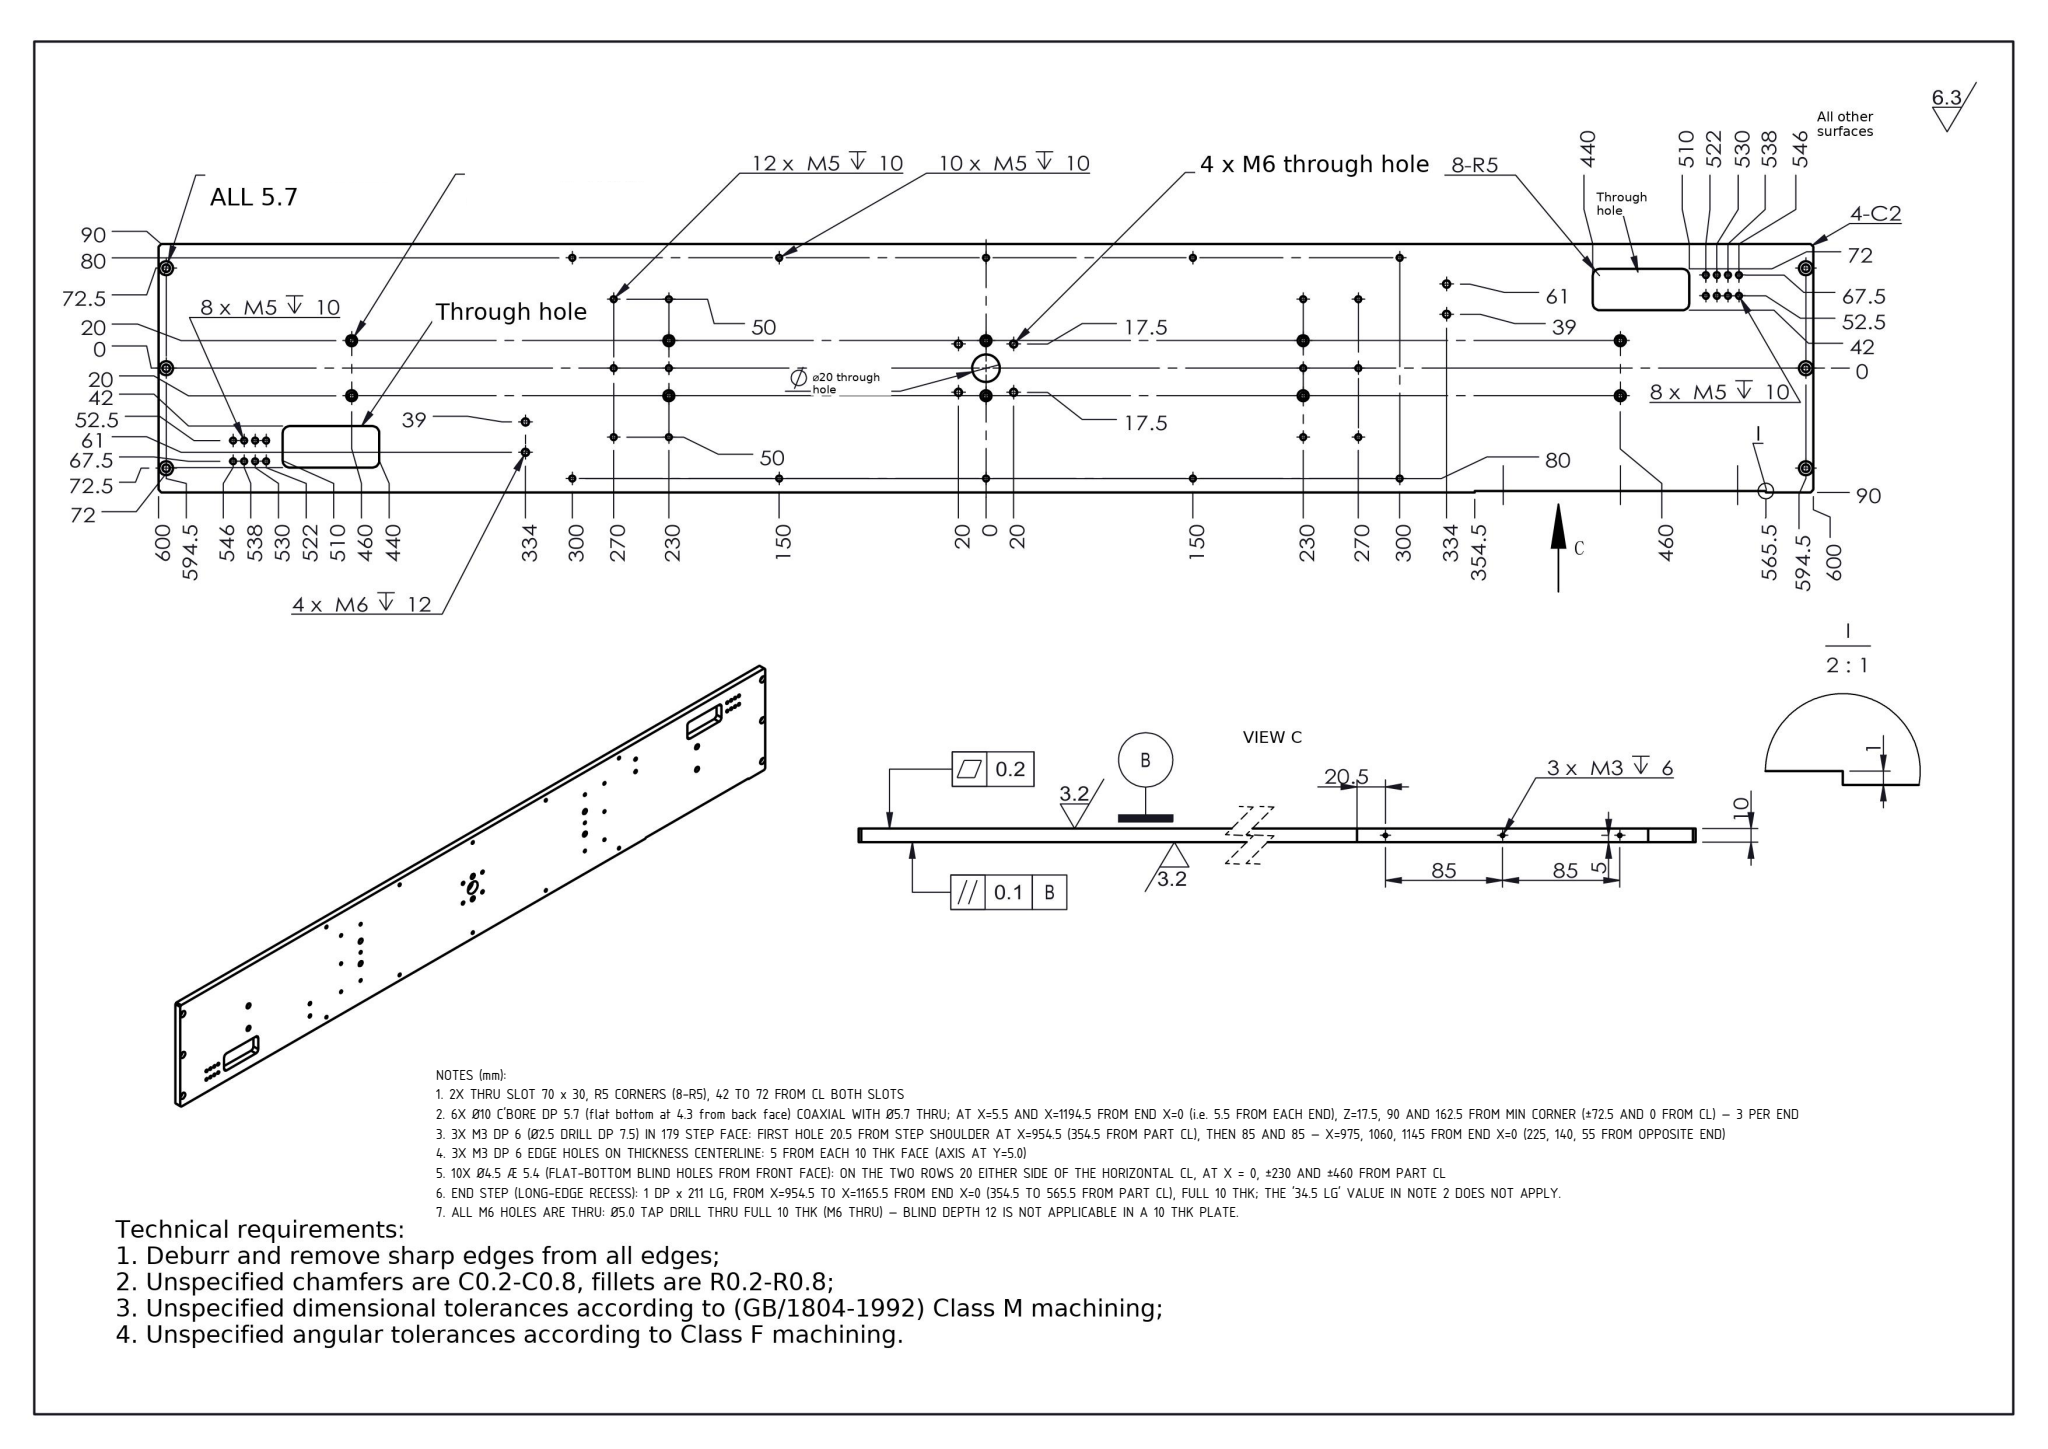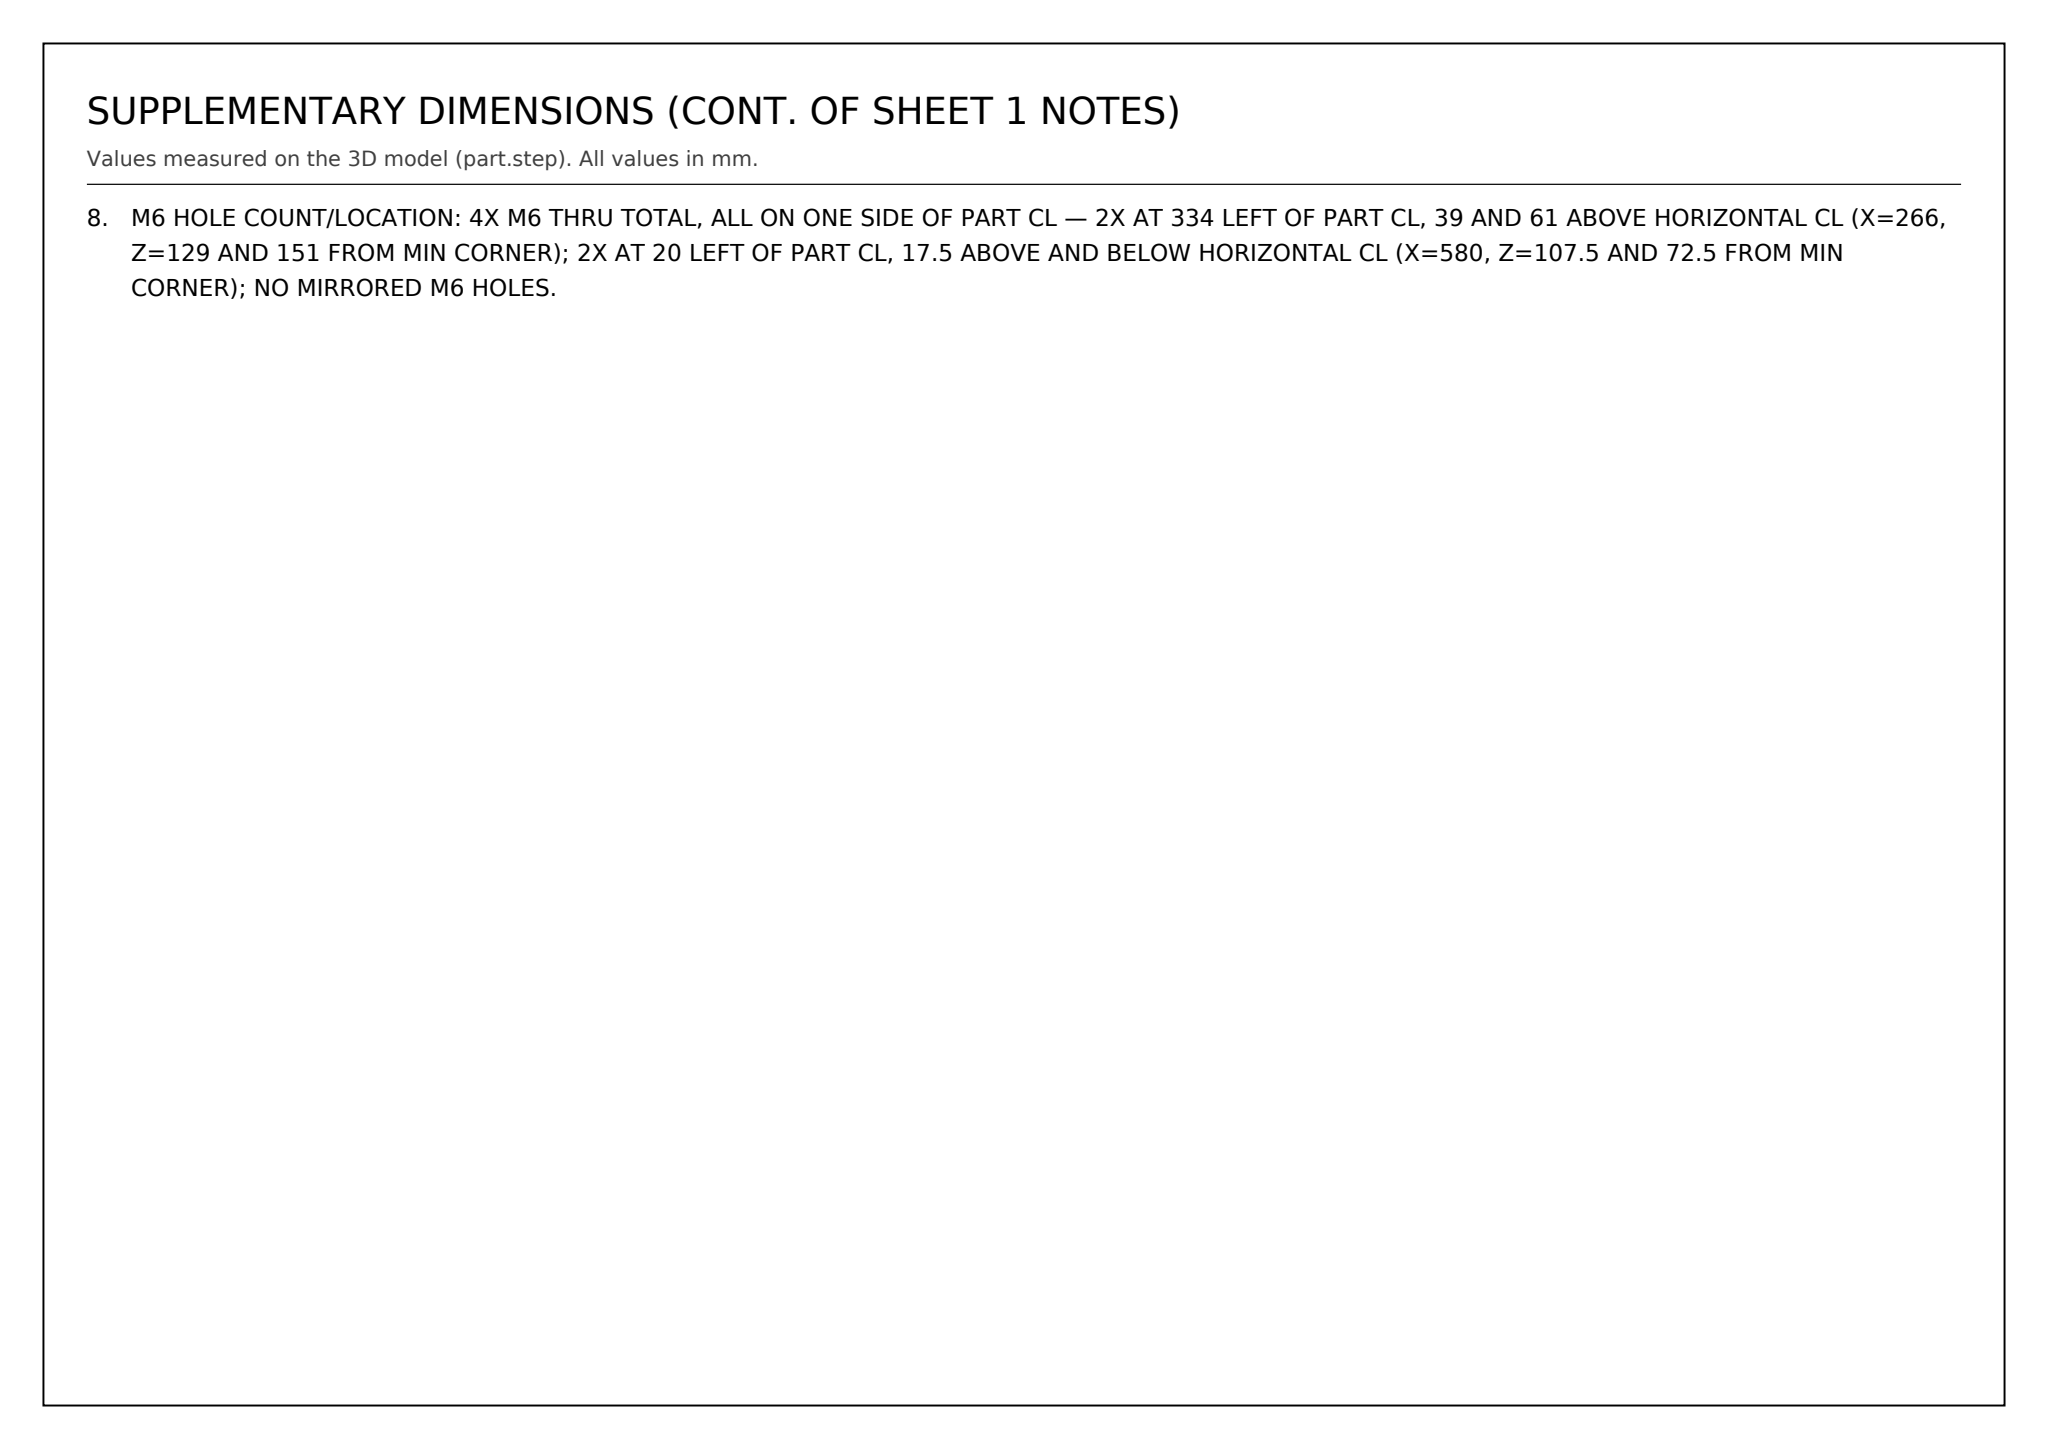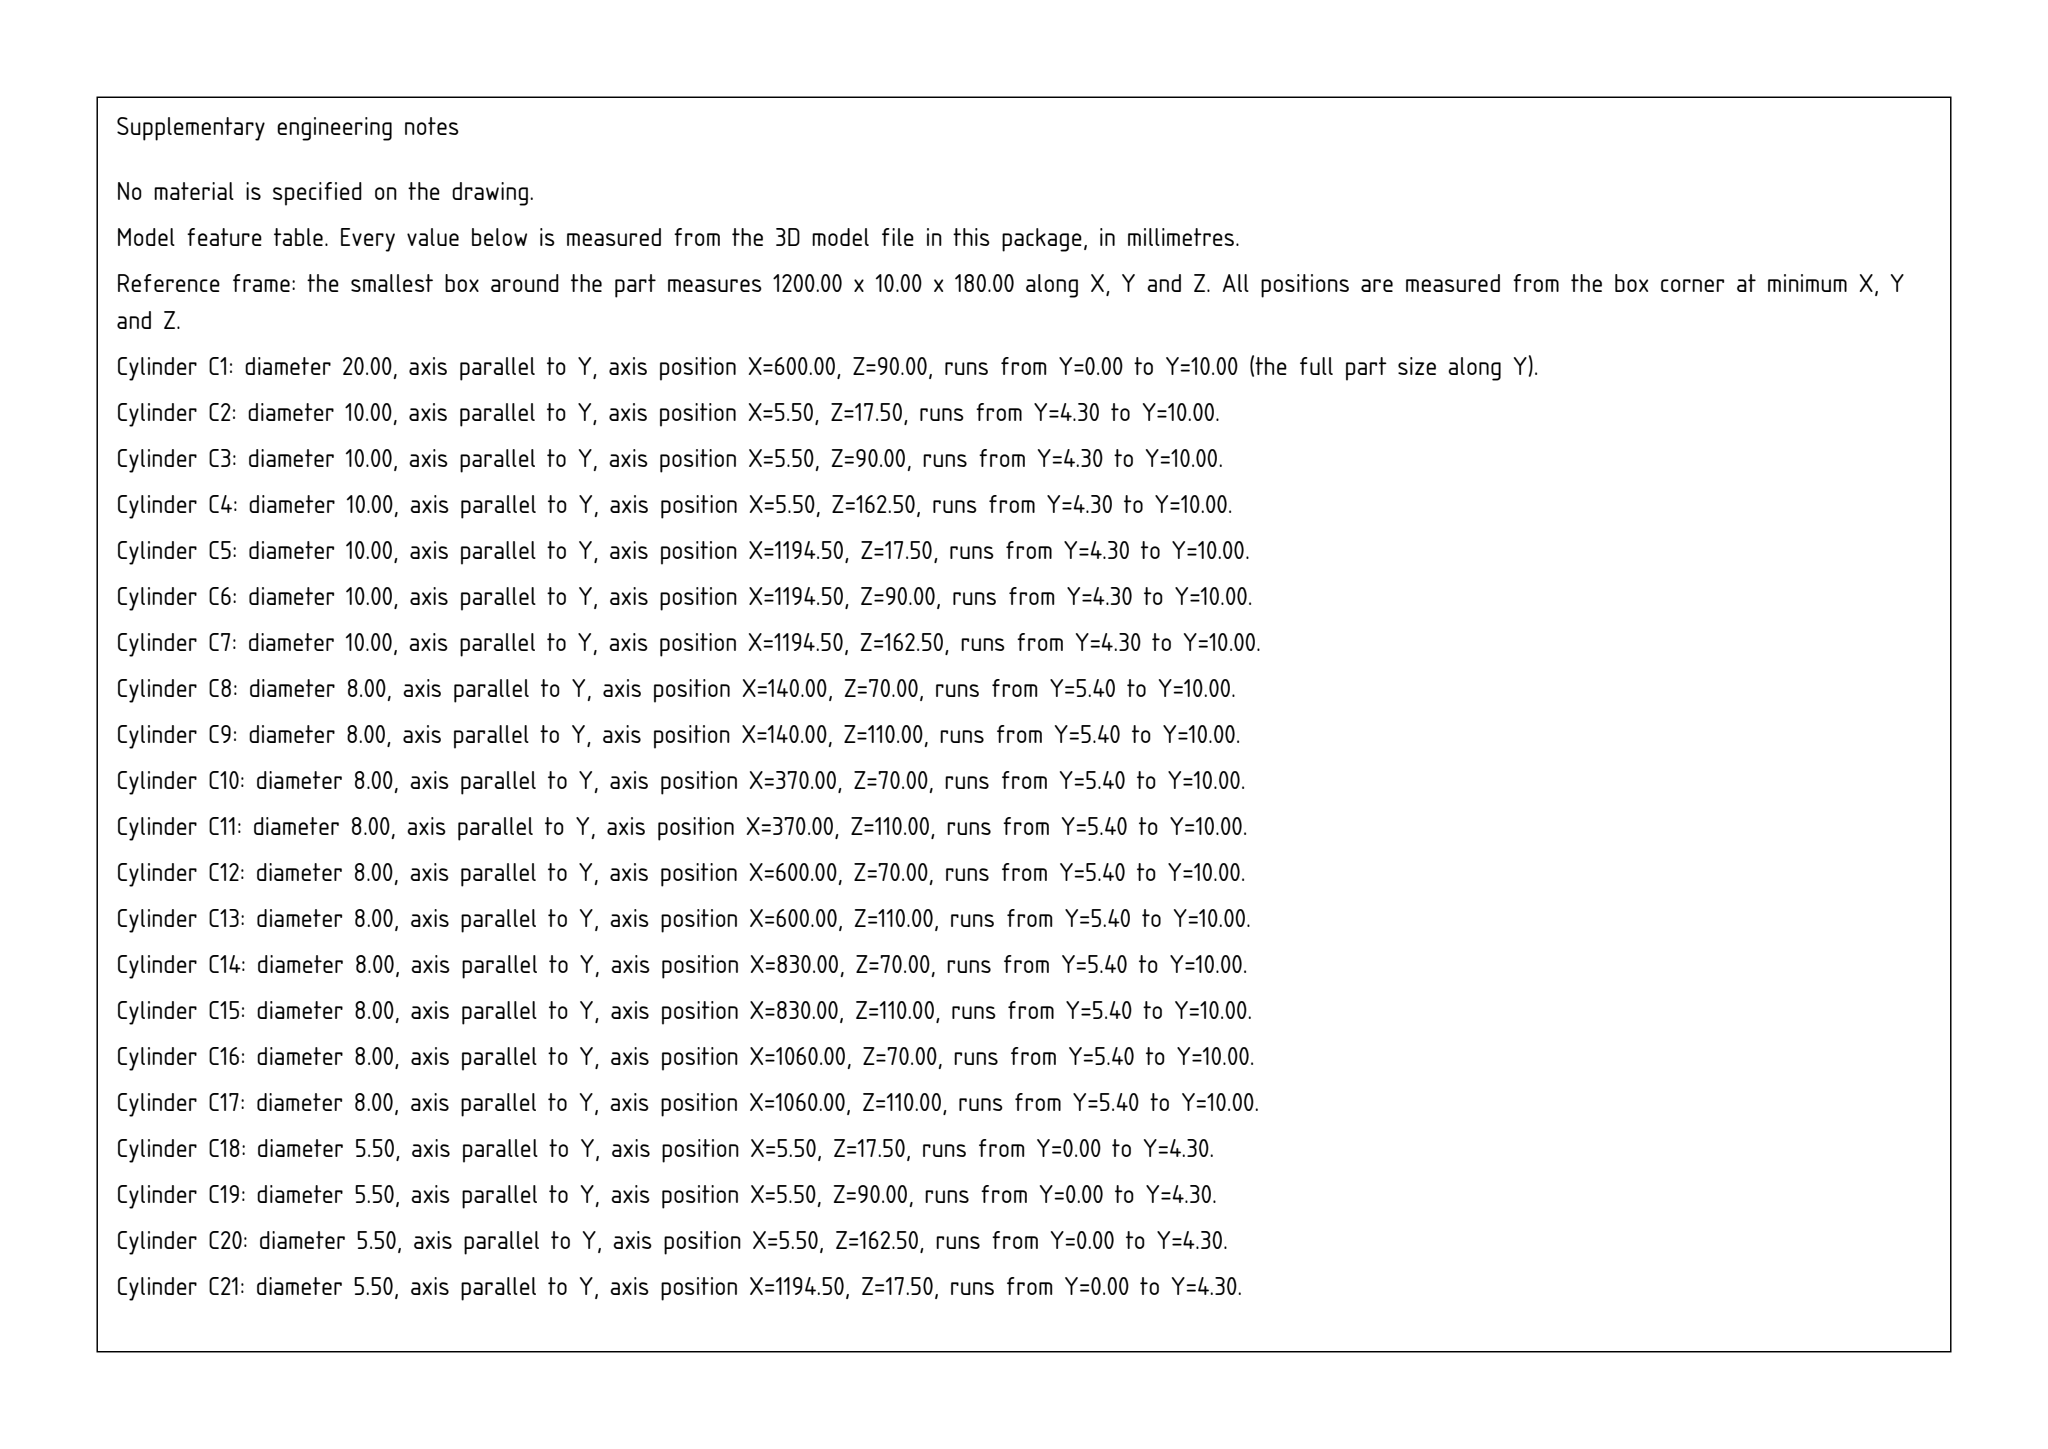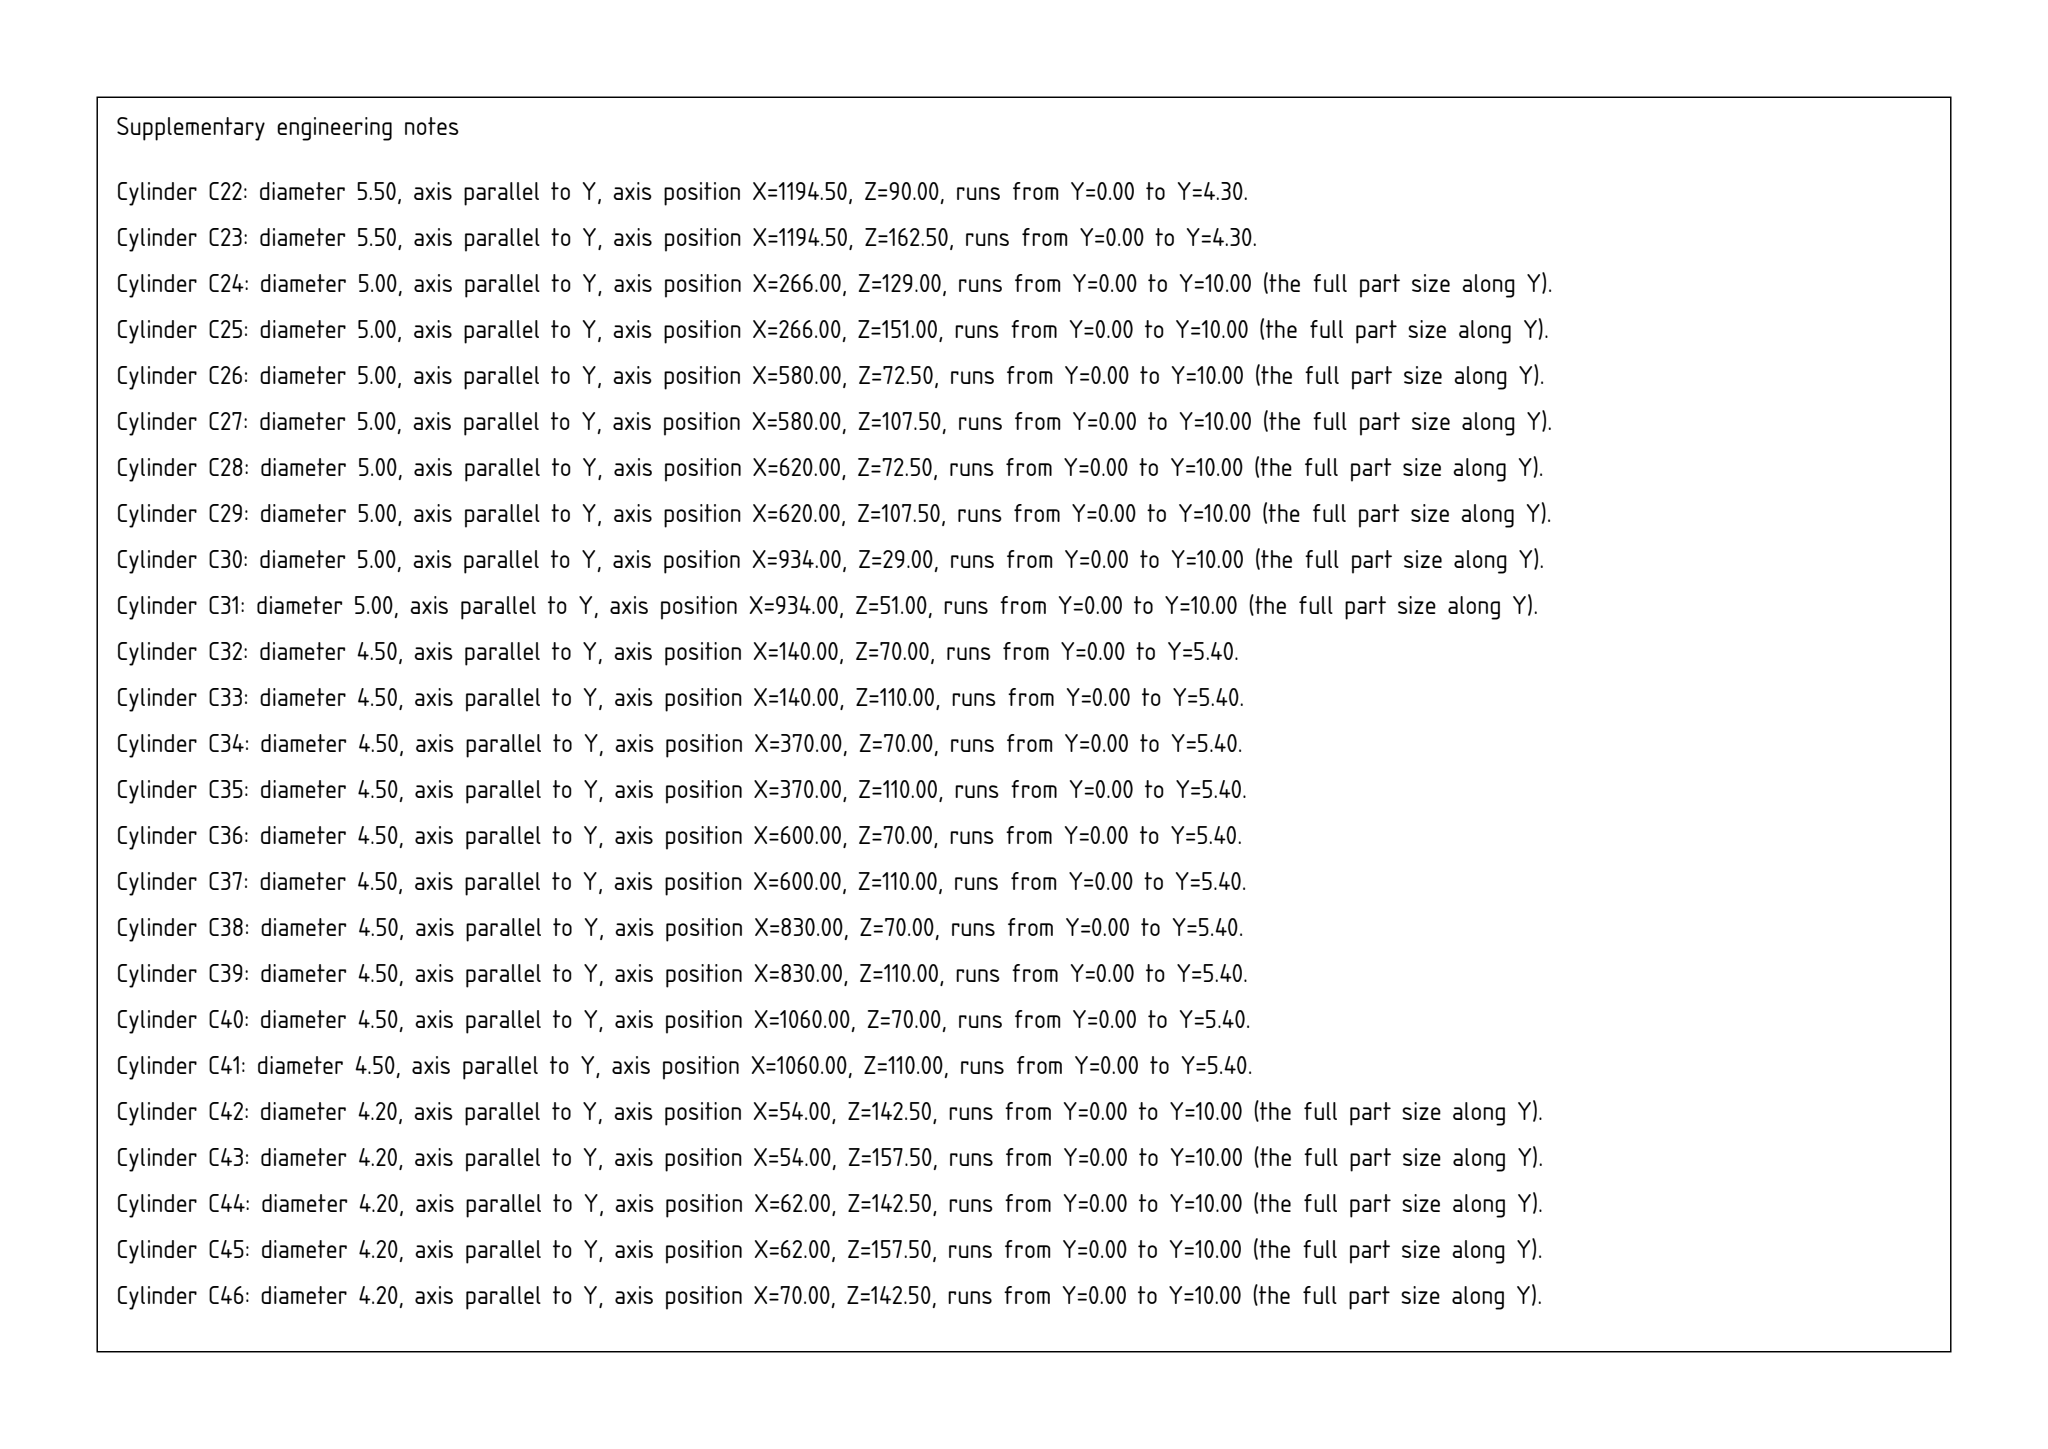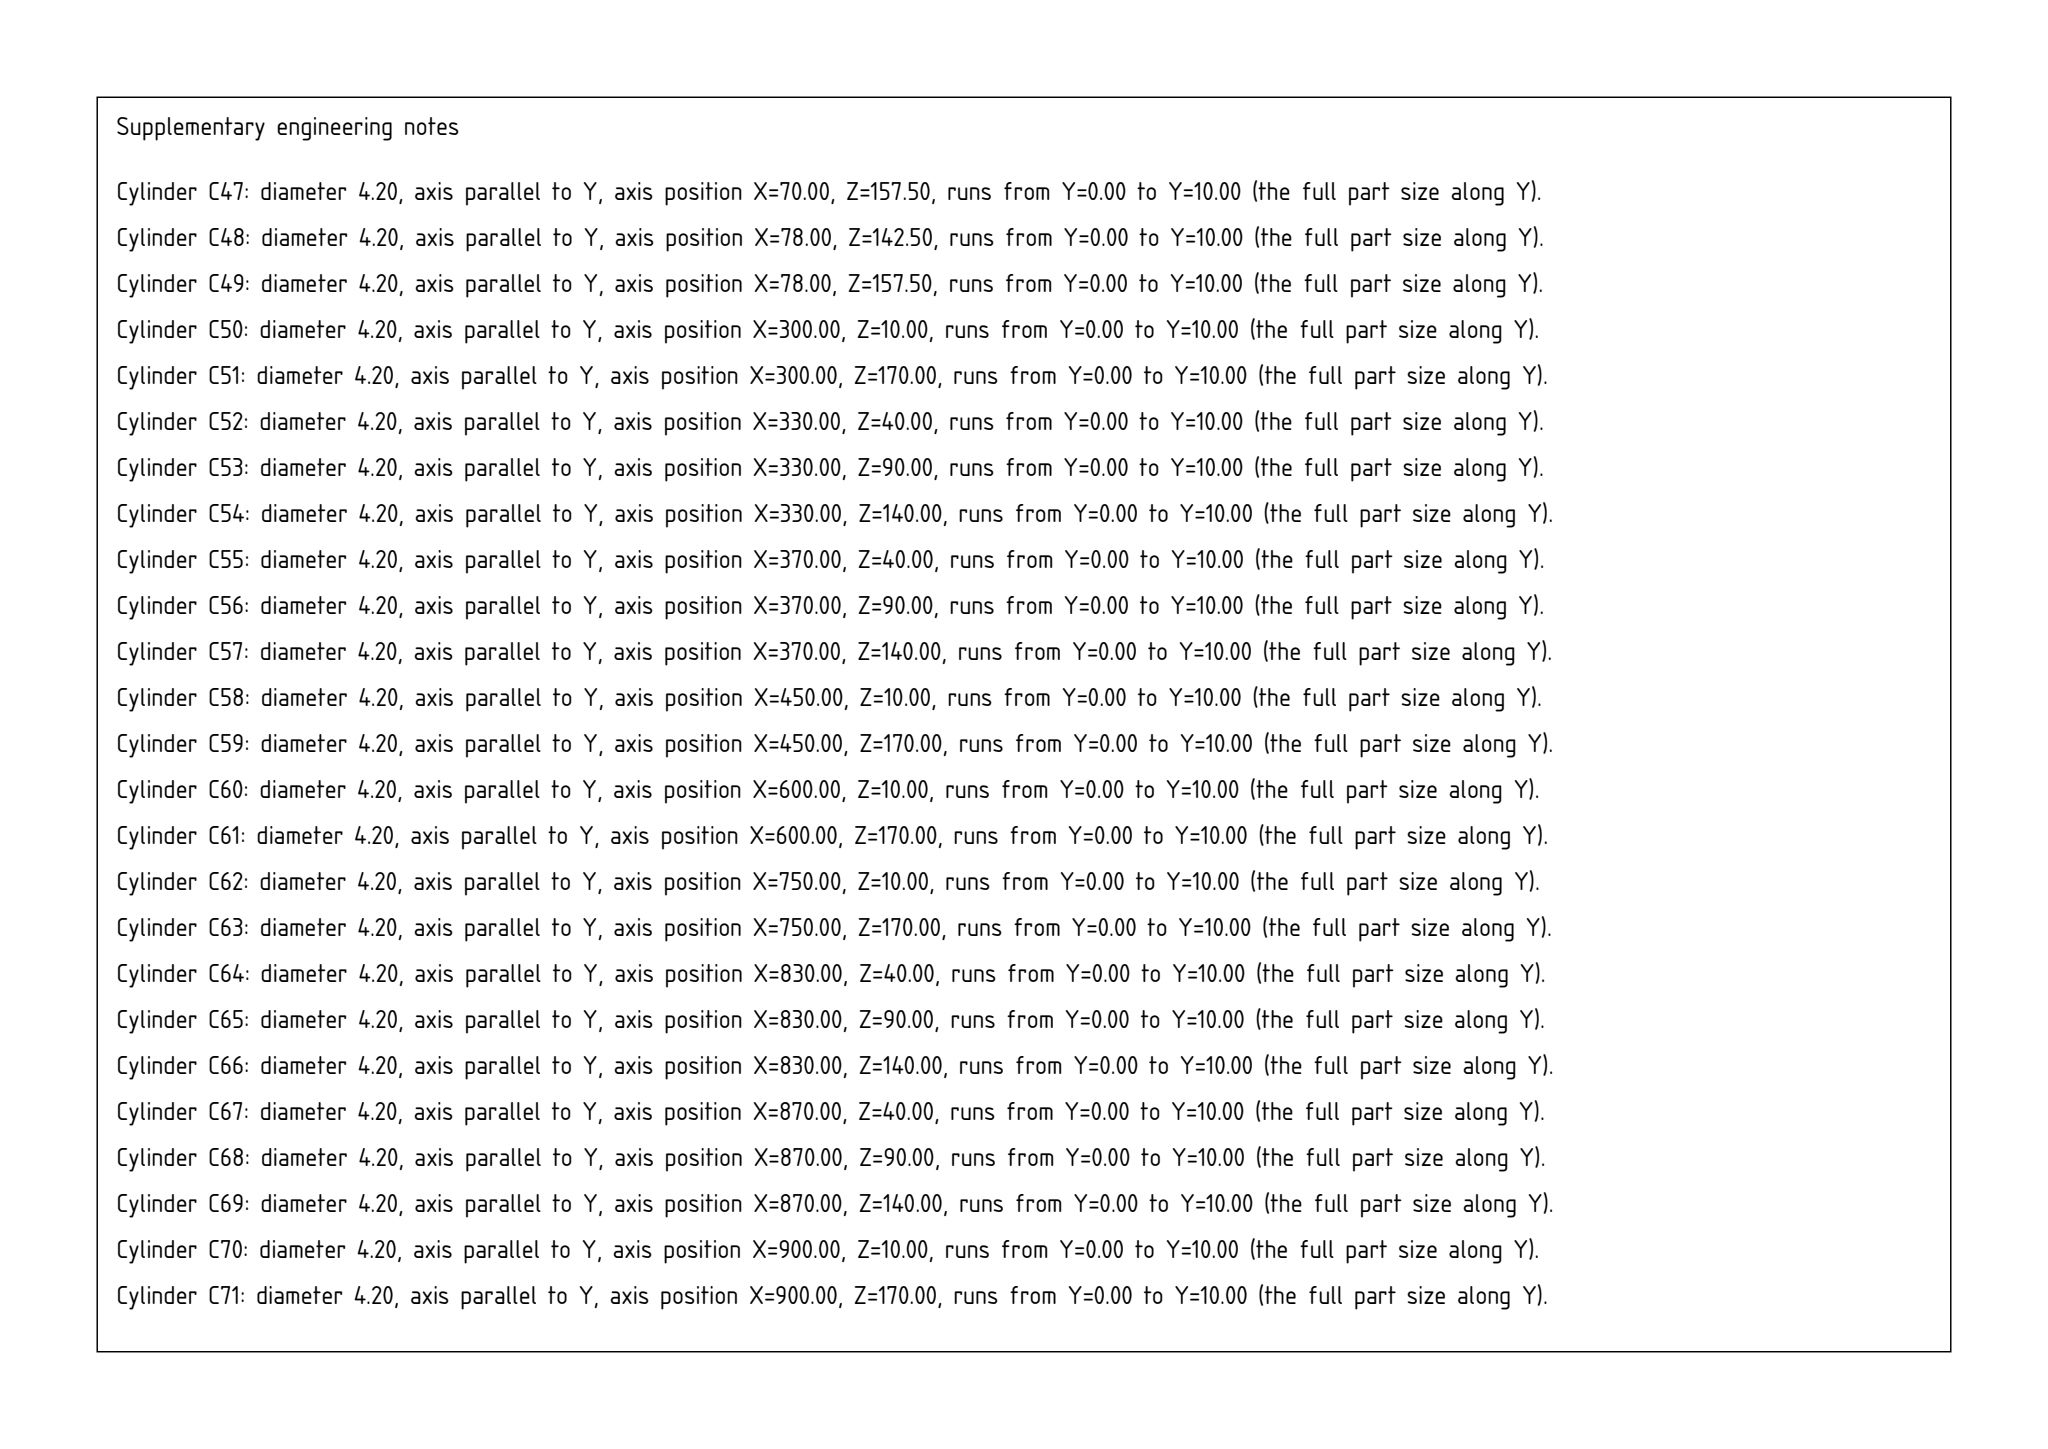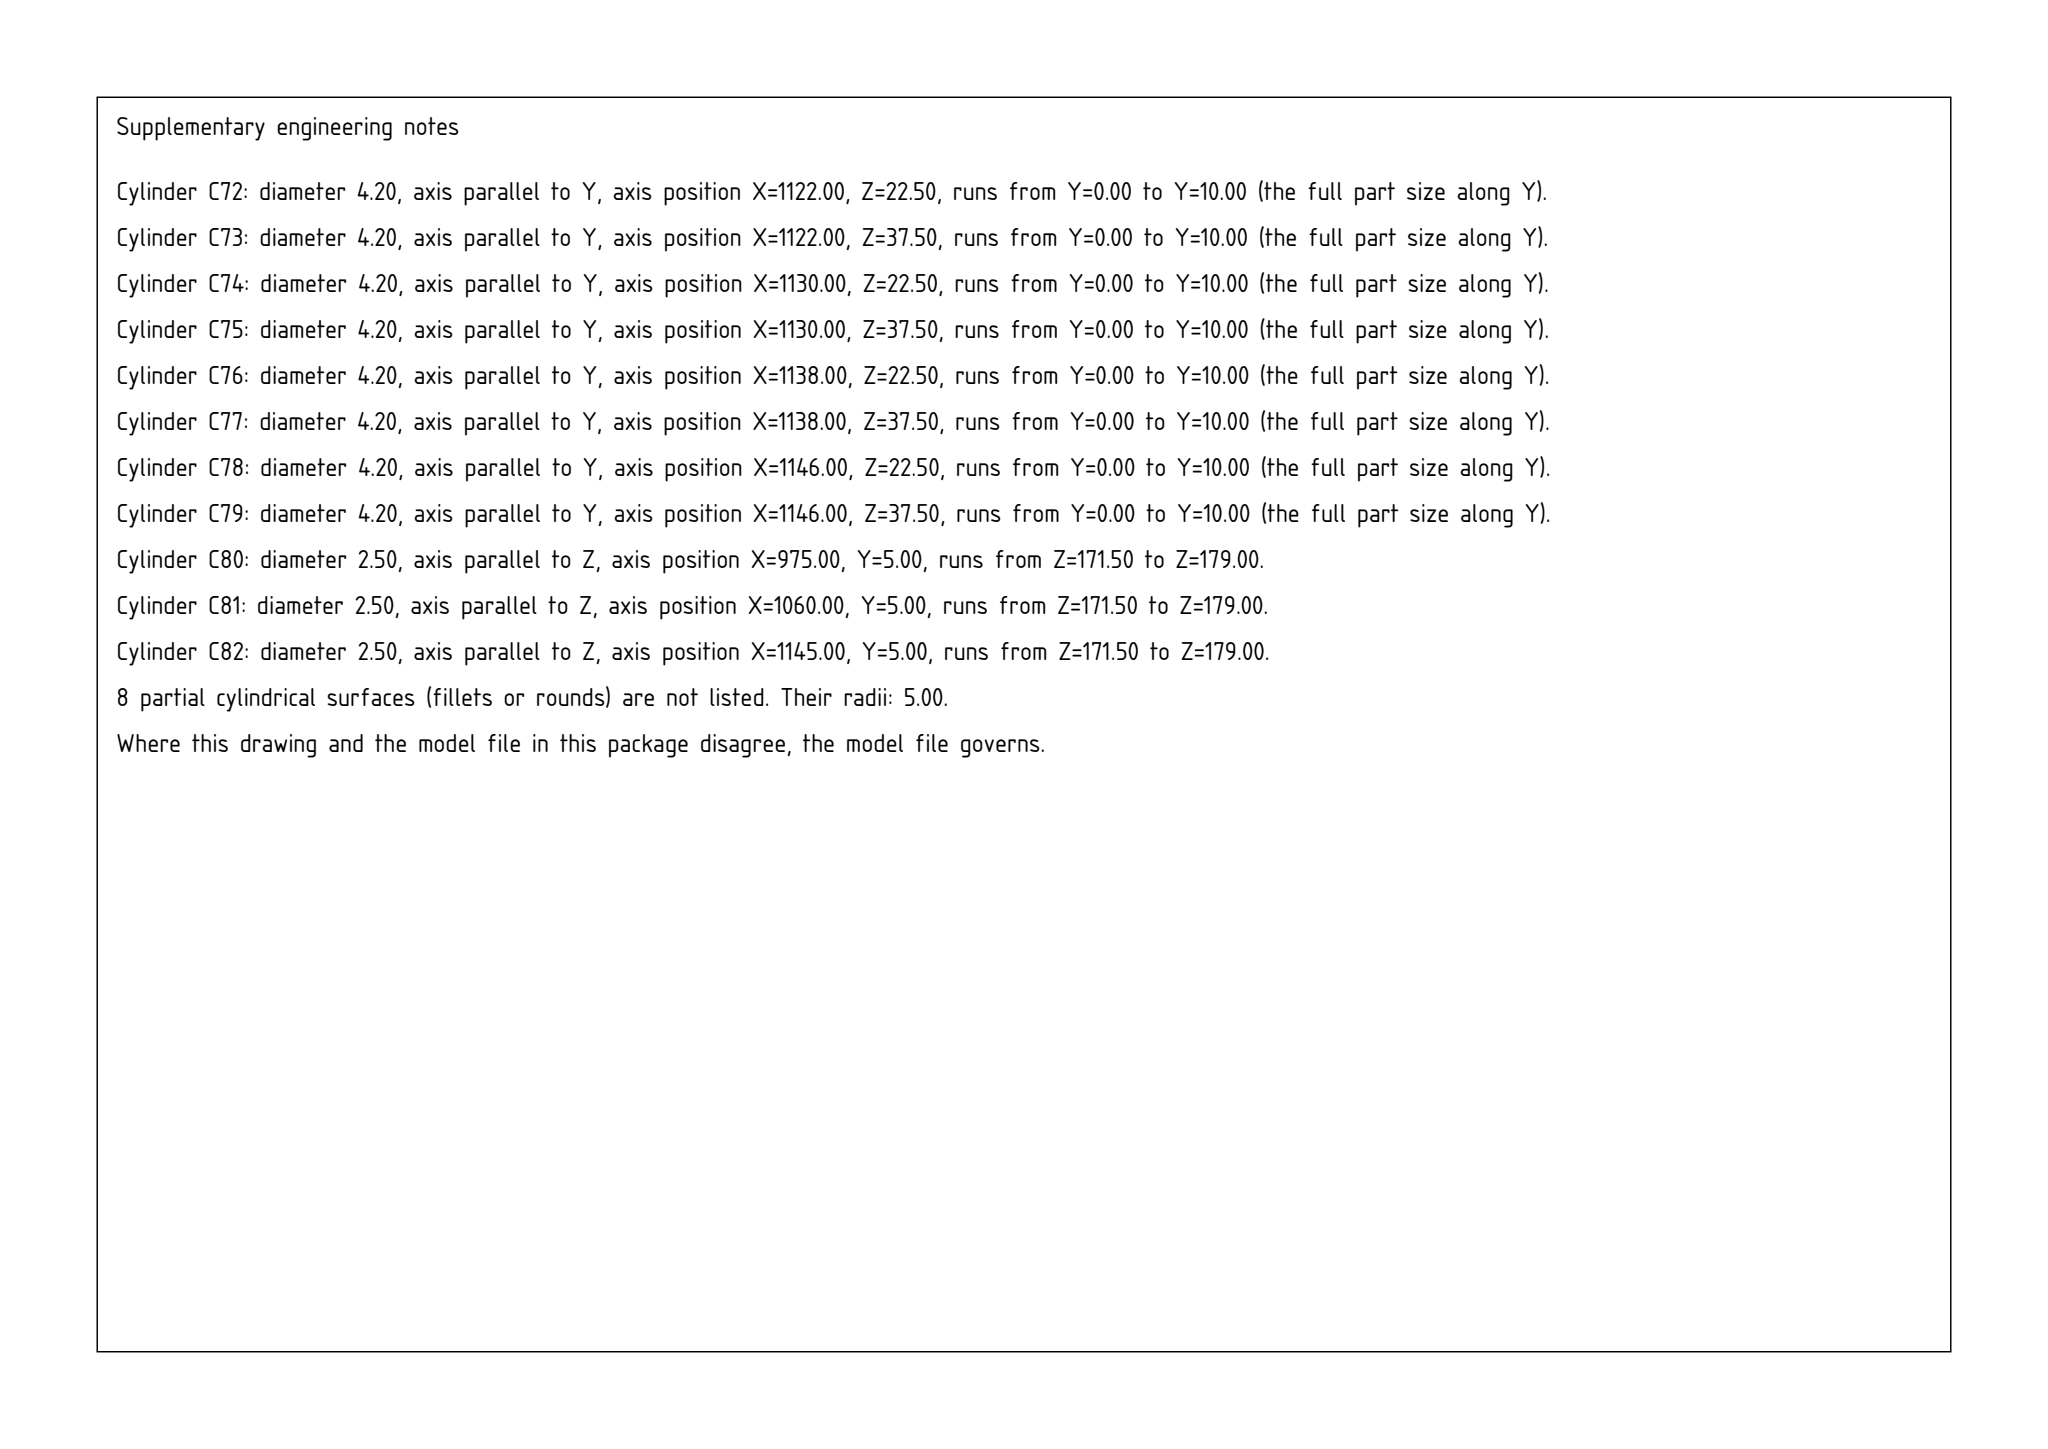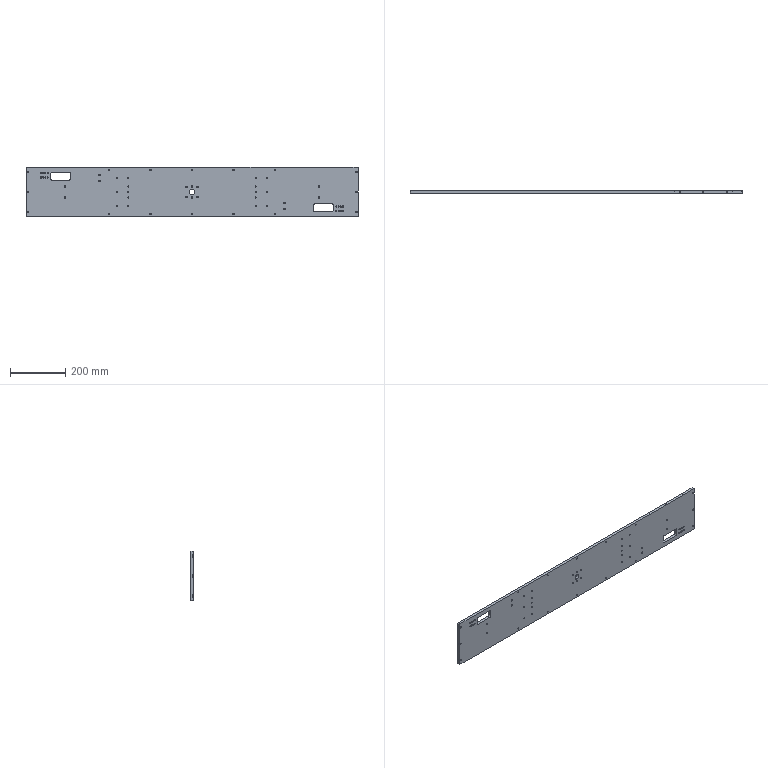Part | SolidWorks | mm | 1 solid | 216 faces | box 1200 x 10 x 180 mm | volume 2099678 mm3 | cylinder 172 | plane 38 | cone 6 | commonest cylinder face diameters 4.2 x76 8 x20 4.5 x20 10 x20 5 x16 5.5 x12 2.5 x6 20 x2
Drawing notes:
2X THRU SLOT 70 x 30, R5 CORNERS (8-R5), 42 TO 72 FROM CL BOTH SLOTS | from the solid: Slot faces x=90/160 & z=132/162 (left), x=1040/1110 & z=18/48 (right); corner cyl Ø10 at (95,137),(95,157) => 70 x 30, R5; z planes 30 apart, ±42 to ±72 from CL z=90
6X Ø10 C'BORE DP 5.7 (flat bottom at 4.3 from back face) COAXIAL WITH Ø5.7 THRU; AT X=5.5 AND X=1194.5 FROM END X=0 (i.e. 5.5 FROM EACH END), Z=17.5, 90 AND 162.5 FROM MIN CORNER (±72.5 AND 0 FROM CL) — 3 PER END | from the solid: Ø10 bores, axis y, from y=4.3 to y=10 (5.7 deep, flat bottom plane y=4.3, area 55 => Ø5.7 thru at centre) at x=5.5 and x=1194.5, z=17.5 / 90 / 162.5; no Ø10 bores at x=594.5 or 605.5
3X M3 DP 6 (Ø2.5 DRILL DP 7.5) IN 179 STEP FACE: FIRST HOLE 20.5 FROM STEP SHOULDER AT X=954.5 (354.5 FROM PART CL), THEN 85 AND 85 — X=975, 1060, 1145 FROM END X=0 (225, 140, 55 FROM OPPOSITE END) | from the solid: cylinders hole/bore dia 2.5 axis z at x=975.0, 1060.0, 1145.0 from z 171.5 to 179.0; axis_plane x=954.5 and z=179.0 extent x[954.5,1165.5] define step shoulder
3X M3 DP 6 EDGE HOLES ON THICKNESS CENTERLINE: 5 FROM EACH 10 THK FACE (AXIS AT Y=5.0) | from the solid: cylinders hole/bore dia 2.5 axis z at y=5.0 with part faces axis_planes y=0.0 and y=10.0
10X Ø4.5 Æ 5.4 (FLAT-BOTTOM BLIND HOLES FROM FRONT FACE): ON THE TWO ROWS 20 EITHER SIDE OF THE HORIZONTAL CL, AT X = 0, ±230 AND ±460 FROM PART CL | from the solid: cylinders kind=hole/bore dia 4.5 axis y at [140,-,70], [140,-,110], [370,-,70], [370,-,110], [600,-,70], [600,-,110], [830,-,70], [830,-,110], [1060,-,70], [1060,-,110], from 0.0 to 5.4 (part CL at x=600, z=90); flat bottoms = axis_planes y=5.4 with 8x8 extents at same x/z
END STEP (LONG-EDGE RECESS): 1 DP x 211 LG, FROM X=954.5 TO X=1165.5 FROM END X=0 (354.5 TO 565.5 FROM PART CL), FULL 10 THK; THE '34.5 LG' VALUE IN NOTE 2 DOES NOT APPLY. | from the solid: plane z=179 extent x[954.5,1165.5] y[0,10] between z=180 faces x[2,954.5] and x[1165.5,1198]; end x-planes at x=954.5 and x=1165.5 extent z[179,180]
ALL M6 HOLES ARE THRU: Ø5.0 TAP DRILL THRU FULL 10 THK (M6 THRU) — BLIND DEPTH 12 IS NOT APPLICABLE IN A 10 THK PLATE. | from the solid: cylinders kind hole/bore dia 5.0, axis y, from 0.0 to 10.0 (4 off)
M6 HOLE COUNT/LOCATION: 4X M6 THRU TOTAL, ALL ON ONE SIDE OF PART CL — 2X AT 334 LEFT OF PART CL, 39 AND 61 ABOVE HORIZONTAL CL (X=266, Z=129 AND 151 FROM MIN CORNER); 2X AT 20 LEFT OF PART CL, 17.5 ABOVE AND BELOW HORIZONTAL CL (X=580, Z=107.5 AND 72.5 FROM MIN CORNER); NO MIRRORED M6 HOLES. | from the solid: cylinders dia 5.0 axis y at [266,null,129], [266,null,151], [580,null,107.5], [580,null,72.5], from 0.0 to 10.0
build123d program:
from build123d import *

# Parameters (mm, degrees)
SKETCH1_W                                            = 1200
SKETCH1_H                                            = 180
BOSS_EXTRUDE1_DEPTH                                  = 5
M6_TAPPED_HOLE1_D                                    = 5
CHAMFER1_SIZE                                        = 2
SKETCH29_W                                           = 70
SKETCH29_H                                           = 30
CUT_EXTRUDE1_DEPTH                                   = 607.795
FILLET1_R                                            = 5
HOLE_SIZE_ACCORDING_TO_HEXAGON_SOCKET_HE_D           = 5.5
HOLE_SIZE_ACCORDING_TO_HEXAGON_SOCKET_HE_CBORE_D     = 10
HOLE_SIZE_ACCORDING_TO_HEXAGON_SOCKET_HE_CBORE_DEPTH = 5.7
M5_TAPPED_HOLE1_AT_2_COUNT                           = 2
M5_TAPPED_HOLE1_AT_2_PITCH                           = 160
LPATTERN1_COUNT                                      = 5
LPATTERN1_PITCH                                      = 150
M5_TAPPED_HOLE2_D                                    = 4.2
M5_TAPPED_HOLE2_DEPTH                                = 12.4
M5_TAPPED_HOLE2_TIP                                  = 1.262
SKETCH36_R                                           = 10
CUT_EXTRUDE2_DEPTH                                   = 607.795
M6_TAPPED_HOLE2_D                                    = 5
M6_TAPPED_HOLE2_DEPTH                                = 15
M6_TAPPED_HOLE2_TIP                                  = 1.502
M5_TAPPED_HOLE3_AT_2_COUNT                           = 2
M5_TAPPED_HOLE3_AT_2_PITCH                           = 15
M5_TAPPED_HOLE4_AT_2_COUNT                           = 2
M5_TAPPED_HOLE4_AT_2_PITCH                           = 15
HOLE_SIZE_ACCORDING_TO_HEXAGON_SOCKE_2_D             = 4.5
HOLE_SIZE_ACCORDING_TO_HEXAGON_SOCKE_2_CBORE_D       = 8
HOLE_SIZE_ACCORDING_TO_HEXAGON_SOCKE_2_CBORE_DEPTH   = 4.6
LPATTERN2_COUNT                                      = 3
LPATTERN2_PITCH                                      = 230
LPATTERN2_COL_COUNT                                  = 3
LPATTERN2_COL_PITCH                                  = 230
SKETCH48_W                                           = 211
SKETCH48_H                                           = 10
CUT_EXTRUDE4_DEPTH                                   = 1
M3_TAPPED_HOLE1_D                                    = 2.5
M3_TAPPED_HOLE1_DEPTH                                = 7.5
M3_TAPPED_HOLE1_TIP                                  = 0.7511
LPATTERN3_COUNT                                      = 4
LPATTERN3_PITCH                                      = 8
LPATTERN4_COUNT                                      = 4
LPATTERN4_PITCH                                      = 8


with BuildPart() as part:
    # Sketch1 → Boss-Extrude1 (new, symmetric)
    with BuildSketch(Plane(origin=(0, 0, 0), x_dir=(1, 0, 0), z_dir=(0, 1, 0))):
        Rectangle(SKETCH1_W, SKETCH1_H)
    extrude(amount=BOSS_EXTRUDE1_DEPTH, both=True)

    # M6 Tapped Hole1 (through all)
    with Locations(Plane(origin=(0, 5, 0), x_dir=(1, 0, 0), z_dir=(0, 1, 0))):
        with Locations((20, 17.5), (-20, 17.5), (-20, -17.5), (20, -17.5)):
            Hole(M6_TAPPED_HOLE1_D / 2)

    # Chamfer1
    chamfer1_edges = [part.edges().sort_by_distance(p)[0] for p in [
        (-600, 0, -90),
        (600, 0, -90),
        (600, 0, 90),
        (-600, 0, 90),
    ]]
    chamfer(chamfer1_edges, length=CHAMFER1_SIZE)

    # Sketch29 → Cut-Extrude1 (cut, through all)
    with BuildSketch(Plane(origin=(0, 5, 0), x_dir=(1, 0, 0), z_dir=(0, 1, 0))):
        with Locations((-475, -57)):
            Rectangle(SKETCH29_W, SKETCH29_H)
        with Locations((475, 57)):
            Rectangle(SKETCH29_W, SKETCH29_H)
    extrude(amount=-CUT_EXTRUDE1_DEPTH, mode=Mode.SUBTRACT)

    # Fillet1
    fillet1_edges = [part.edges().sort_by_distance(p)[0] for p in [
        (-510, 0, 72),
        (-510, 0, 42),
        (-440, 0, 42),
        (-440, 0, 72),
        (440, 0, -42),
        (440, 0, -72),
        (510, 0, -72),
        (510, 0, -42),
    ]]
    fillet(fillet1_edges, radius=FILLET1_R)

    # Hole Size according to Hexagon Socket He (through all)
    with Locations(Plane(origin=(0, 5, 0), x_dir=(1, 0, 0), z_dir=(0, 1, 0))):
        with Locations((-594.5, 72.5), (-594.5, 0), (-594.5, -72.5), (594.5, -72.5), (594.5, 0), (594.5, 72.5)):
            CounterBoreHole(HOLE_SIZE_ACCORDING_TO_HEXAGON_SOCKET_HE_D / 2, HOLE_SIZE_ACCORDING_TO_HEXAGON_SOCKET_HE_CBORE_D / 2, HOLE_SIZE_ACCORDING_TO_HEXAGON_SOCKET_HE_CBORE_DEPTH)

    # Sketch32 → M5 Tapped Hole1 (revolve, cut)
    with BuildSketch(Plane(origin=(-300, 5, -80), x_dir=(0, 0, 1), z_dir=(1, 0, 0))):
        Polygon((0, 0), (0, 13.662), (2.1, 12.4), (2.1, 0), align=None)
    m5_tapped_hole1 = revolve(axis=Axis((-300, 11.35, -80), (0, -1, 0)), mode=Mode.SUBTRACT)

    # M5 Tapped Hole1 at 2: M5 Tapped Hole1 ×2
    with Locations(*[(0, 0, i * M5_TAPPED_HOLE1_AT_2_PITCH) for i in range(1, M5_TAPPED_HOLE1_AT_2_COUNT)]):
        add(m5_tapped_hole1, mode=Mode.SUBTRACT)

    # LPattern1: M5 Tapped Hole1 ×5
    with Locations(*[(i * LPATTERN1_PITCH, 0, 0) for i in range(1, LPATTERN1_COUNT)]):
        add(m5_tapped_hole1, mode=Mode.SUBTRACT)

    # LPattern1 copy 1 sketch → LPattern1 copy 1 (revolve, cut)
    with BuildSketch(Plane(origin=(-150, 5, 80), x_dir=(0, 0, 1), z_dir=(1, 0, 0))):
        Polygon((0, 0), (0, 13.662), (2.1, 12.4), (2.1, 0), align=None)
    revolve(axis=Axis((-150, 11.35, 80), (0, -1, 0)), mode=Mode.SUBTRACT)

    # LPattern1 copy 2 sketch → LPattern1 copy 2 (revolve, cut)
    with BuildSketch(Plane(origin=(0, 5, 80), x_dir=(0, 0, 1), z_dir=(1, 0, 0))):
        Polygon((0, 0), (0, 13.662), (2.1, 12.4), (2.1, 0), align=None)
    revolve(axis=Axis((0, 11.35, 80), (0, -1, 0)), mode=Mode.SUBTRACT)

    # LPattern1 copy 3 sketch → LPattern1 copy 3 (revolve, cut)
    with BuildSketch(Plane(origin=(150, 5, 80), x_dir=(0, 0, 1), z_dir=(1, 0, 0))):
        Polygon((0, 0), (0, 13.662), (2.1, 12.4), (2.1, 0), align=None)
    revolve(axis=Axis((150, 11.35, 80), (0, -1, 0)), mode=Mode.SUBTRACT)

    # LPattern1 copy 4 sketch → LPattern1 copy 4 (revolve, cut)
    with BuildSketch(Plane(origin=(300, 5, 80), x_dir=(0, 0, 1), z_dir=(1, 0, 0))):
        Polygon((0, 0), (0, 13.662), (2.1, 12.4), (2.1, 0), align=None)
    revolve(axis=Axis((300, 11.35, 80), (0, -1, 0)), mode=Mode.SUBTRACT)

    # M5 Tapped Hole2
    with Locations(Plane(origin=(0, 5, 0), x_dir=(1, 0, 0), z_dir=(0, 1, 0))):
        with Locations((-270, 50), (-270, 0), (-230, 50), (-230, 0), (-230, -50), (-270, -50), (270, -50), (230, -50), (230, 0), (230, 50), (270, 0), (270, 50)):
            Hole(M5_TAPPED_HOLE2_D / 2, depth=M5_TAPPED_HOLE2_DEPTH)
            with Locations((0, 0, -(M5_TAPPED_HOLE2_DEPTH + M5_TAPPED_HOLE2_TIP / 2))):  # 118° drill point
                Cone(0, M5_TAPPED_HOLE2_D / 2, M5_TAPPED_HOLE2_TIP, mode=Mode.SUBTRACT)

    # Sketch36 → Cut-Extrude2 (cut, through all)
    with BuildSketch(Plane(origin=(0, 5, 0), x_dir=(1, 0, 0), z_dir=(0, 1, 0))):
        with Locations(Location((0, 0, 0), (0, 0, 270))):
            Circle(SKETCH36_R)
    extrude(amount=-CUT_EXTRUDE2_DEPTH, mode=Mode.SUBTRACT)

    # M6 Tapped Hole2
    with Locations(Plane(origin=(0, 5, 0), x_dir=(1, 0, 0), z_dir=(0, 1, 0))):
        with Locations((-334, -39), (-334, -61), (334, 61), (334, 39)):
            Hole(M6_TAPPED_HOLE2_D / 2, depth=M6_TAPPED_HOLE2_DEPTH)
            with Locations((0, 0, -(M6_TAPPED_HOLE2_DEPTH + M6_TAPPED_HOLE2_TIP / 2))):  # 118° drill point
                Cone(0, M6_TAPPED_HOLE2_D / 2, M6_TAPPED_HOLE2_TIP, mode=Mode.SUBTRACT)

    # Sketch39 → M5 Tapped Hole3 (revolve, cut)
    with BuildSketch(Plane(origin=(-522, 5, 52.5), x_dir=(0, 0, 1), z_dir=(1, 0, 0))):
        Polygon((0, 0), (0, 13.662), (2.1, 12.4), (2.1, 0), align=None)
    m5_tapped_hole3 = revolve(axis=Axis((-522, 11.35, 52.5), (0, -1, 0)), mode=Mode.SUBTRACT)

    # M5 Tapped Hole3 at 2: M5 Tapped Hole3 ×2
    with Locations(*[(0, 0, i * M5_TAPPED_HOLE3_AT_2_PITCH) for i in range(1, M5_TAPPED_HOLE3_AT_2_COUNT)]):
        add(m5_tapped_hole3, mode=Mode.SUBTRACT)

    # Sketch41 → M5 Tapped Hole4 (revolve, cut)
    with BuildSketch(Plane(origin=(522, 5, -67.5), x_dir=(0, 0, 1), z_dir=(1, 0, 0))):
        Polygon((0, 0), (0, 13.662), (2.1, 12.4), (2.1, 0), align=None)
    m5_tapped_hole4 = revolve(axis=Axis((522, 11.35, -67.5), (0, -1, 0)), mode=Mode.SUBTRACT)

    # M5 Tapped Hole4 at 2: M5 Tapped Hole4 ×2
    with Locations(*[(0, 0, i * M5_TAPPED_HOLE4_AT_2_PITCH) for i in range(1, M5_TAPPED_HOLE4_AT_2_COUNT)]):
        add(m5_tapped_hole4, mode=Mode.SUBTRACT)

    # Hole Size according to Hexagon Socke 2 (through all)
    with Locations(Plane(origin=(0, 5, 0), x_dir=(1, 0, 0), z_dir=(0, 1, 0))):
        with Locations((0, 20), (0, -20)):
            hole_size_according_to_hexagon_socke_2 = CounterBoreHole(HOLE_SIZE_ACCORDING_TO_HEXAGON_SOCKE_2_D / 2, HOLE_SIZE_ACCORDING_TO_HEXAGON_SOCKE_2_CBORE_D / 2, HOLE_SIZE_ACCORDING_TO_HEXAGON_SOCKE_2_CBORE_DEPTH)

    # LPattern2: Hole Size according to Hexagon Socke 2 ×3
    with Locations(*[(i * LPATTERN2_PITCH, 0, 0) for i in range(1, LPATTERN2_COUNT)]):
        add(hole_size_according_to_hexagon_socke_2, mode=Mode.SUBTRACT)

    # LPattern2 col: Hole Size according to Hexagon Socke 2 ×3
    with Locations(*[(-i * LPATTERN2_COL_PITCH, 0, 0) for i in range(1, LPATTERN2_COL_COUNT)]):
        add(hole_size_according_to_hexagon_socke_2, mode=Mode.SUBTRACT)

    # Sketch48 → Cut-Extrude4 (cut)
    with BuildSketch(Plane.XY.offset(90)):
        with Locations((460, 0)):
            Rectangle(SKETCH48_W, SKETCH48_H)
    extrude(amount=-CUT_EXTRUDE4_DEPTH, mode=Mode.SUBTRACT)

    # M3 Tapped Hole1
    with Locations(Plane.XY.offset(89)):
        with Locations((545, 0), (460, 0), (375, 0)):
            Hole(M3_TAPPED_HOLE1_D / 2, depth=M3_TAPPED_HOLE1_DEPTH)
            with Locations((0, 0, -(M3_TAPPED_HOLE1_DEPTH + M3_TAPPED_HOLE1_TIP / 2))):  # 118° drill point
                Cone(0, M3_TAPPED_HOLE1_D / 2, M3_TAPPED_HOLE1_TIP, mode=Mode.SUBTRACT)

    # LPattern3: M5 Tapped Hole3 ×4
    with Locations(*[(-i * LPATTERN3_PITCH, 0, 0) for i in range(1, LPATTERN3_COUNT)]):
        add(m5_tapped_hole3, mode=Mode.SUBTRACT)

    # LPattern3 copy 1 sketch → LPattern3 copy 1 (revolve, cut)
    with BuildSketch(Plane(origin=(-530, 5, 67.5), x_dir=(0, 0, 1), z_dir=(1, 0, 0))):
        Polygon((0, 0), (0, 13.662), (2.1, 12.4), (2.1, 0), align=None)
    revolve(axis=Axis((-530, 11.35, 67.5), (0, -1, 0)), mode=Mode.SUBTRACT)

    # LPattern3 copy 2 sketch → LPattern3 copy 2 (revolve, cut)
    with BuildSketch(Plane(origin=(-538, 5, 67.5), x_dir=(0, 0, 1), z_dir=(1, 0, 0))):
        Polygon((0, 0), (0, 13.662), (2.1, 12.4), (2.1, 0), align=None)
    revolve(axis=Axis((-538, 11.35, 67.5), (0, -1, 0)), mode=Mode.SUBTRACT)

    # LPattern3 copy 3 sketch → LPattern3 copy 3 (revolve, cut)
    with BuildSketch(Plane(origin=(-546, 5, 67.5), x_dir=(0, 0, 1), z_dir=(1, 0, 0))):
        Polygon((0, 0), (0, 13.662), (2.1, 12.4), (2.1, 0), align=None)
    revolve(axis=Axis((-546, 11.35, 67.5), (0, -1, 0)), mode=Mode.SUBTRACT)

    # LPattern4: M5 Tapped Hole4 ×4
    with Locations(*[(i * LPATTERN4_PITCH, 0, 0) for i in range(1, LPATTERN4_COUNT)]):
        add(m5_tapped_hole4, mode=Mode.SUBTRACT)

    # LPattern4 copy 1 sketch → LPattern4 copy 1 (revolve, cut)
    with BuildSketch(Plane(origin=(530, 5, -52.5), x_dir=(0, 0, 1), z_dir=(1, 0, 0))):
        Polygon((0, 0), (0, 13.662), (2.1, 12.4), (2.1, 0), align=None)
    revolve(axis=Axis((530, 11.35, -52.5), (0, -1, 0)), mode=Mode.SUBTRACT)

    # LPattern4 copy 2 sketch → LPattern4 copy 2 (revolve, cut)
    with BuildSketch(Plane(origin=(538, 5, -52.5), x_dir=(0, 0, 1), z_dir=(1, 0, 0))):
        Polygon((0, 0), (0, 13.662), (2.1, 12.4), (2.1, 0), align=None)
    revolve(axis=Axis((538, 11.35, -52.5), (0, -1, 0)), mode=Mode.SUBTRACT)

    # LPattern4 copy 3 sketch → LPattern4 copy 3 (revolve, cut)
    with BuildSketch(Plane(origin=(546, 5, -52.5), x_dir=(0, 0, 1), z_dir=(1, 0, 0))):
        Polygon((0, 0), (0, 13.662), (2.1, 12.4), (2.1, 0), align=None)
    revolve(axis=Axis((546, 11.35, -52.5), (0, -1, 0)), mode=Mode.SUBTRACT)


solid = part.part